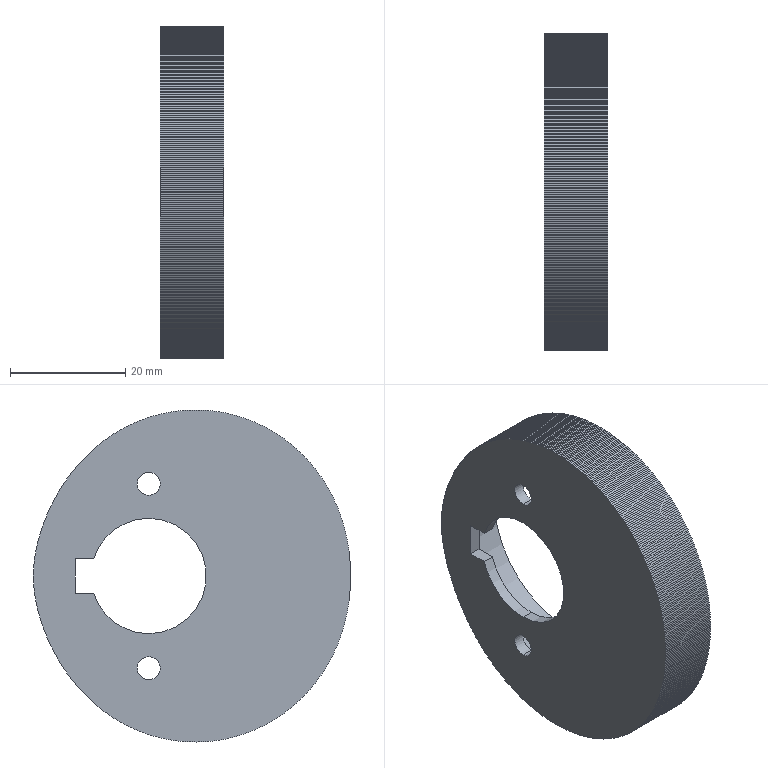Component | SolidWorks | CamGroup4-1_Cam2-1 | 1 solid | 644 faces | volume 17361 mm3 | plane 635 | cylinder 9 | commonest cylinder face diameters 4 x4 20 x3 36 x2